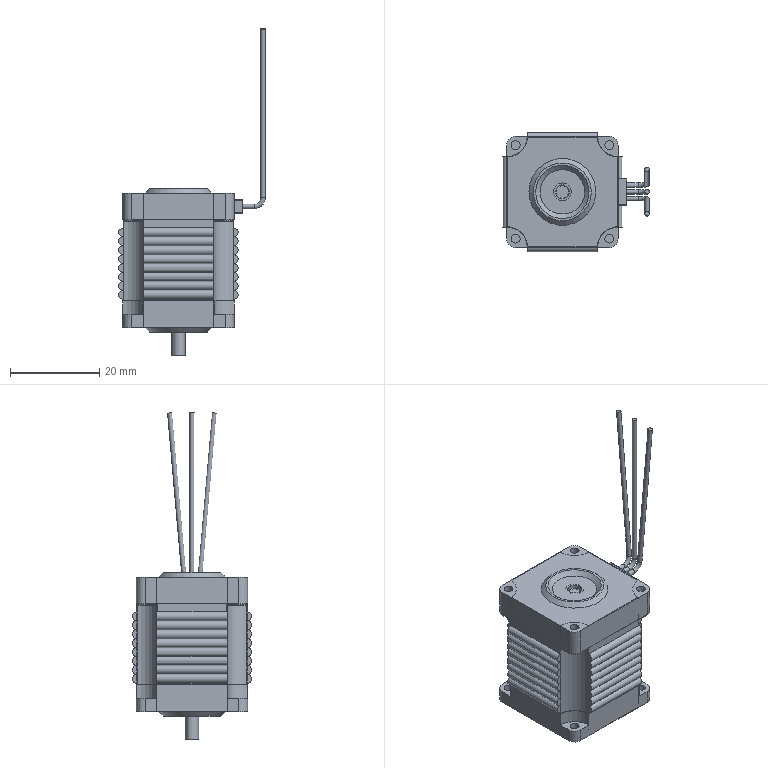Assembly | NX | mm | 8 component files | 8 solids | 300 faces | box 32.9 x 26.8 x 73.5 mm | volume 2197 mm3 | plane 145 | cylinder 119 | cone 19 | torus 10 | sphere 7 | commonest cylinder face diameters 2 x40 0.2 x23 9.2 x16 4 x13 1 x9 3 x5 9.4 x4 9 x4
Bill of materials:
unnamed part 1 | 1 |  | Flat annular ring with a central circular through-hole and small chamfers on the outer edges of both faces.
unnamed part 2 | 1 |  | Open square tray or cup on a rounded-square base flange. There is a through-hole at each of the four corners, and the walls have concave quarter-round notches at the corners next to the holes. The floor has a recessed circular annular groove and a small raised central boss with a through-hole. The underside has a shallow circular chamfered protrusion.
unnamed part 3 | 1 |  | Rounded-square solid block with a through-hole at each of the four corners. On one face is a raised truncated-cone circular boss with an annular recess and a central hole. A small rectangular protrusion sticks out from one side face; it has a recessed rectangular opening containing three small circular holes.
unnamed part 4 | 1 |  | Plain solid straight cylindrical rod with flat ends. It is long compared to its diameter.
unnamed part 5 | 1 |  | Hollow square tube-like shell, open at both ends. Each corner has a concave scalloped channel running its full height. A set of evenly spaced horizontal rounded ribs or rolls covers the middle band of each face, and thin lobed tabs or flanges stick out at the corners near one end.
unnamed part 6 | 3 |  | Thin solid round wire or rod with one bend of roughly 90 degrees near one end, giving a long straight leg and a short straight leg.
Mates:
1. parallel | Stepper_Front 1 face | Stepper_Mid 1 face
2. distance | Stepper_Front 1 face | Stepper_Mid 1 face
3. fix | Stepper_Front 1 component
4. touch align | Stepper_Front 1 face | Stepper_Washer 1 face
5. distance | Stepper_Front 1 face | Stepper_Washer 1 face
6. parallel | Stepper_Back 1 face | Stepper_Front 1 face
7. touch align | Stepper_Mid 1 face | Stepper_Back 1 face
8. touch align | Stepper_Back 1 face | Stepper_Shaft 1 face
9. distance | Stepper_Back 1 face | Stepper_Shaft 1 face
10. distance | Stepper_Mid 1 face | Stepper_Front 1 face
11. concentric | Stepper_Wire 3 edge | Stepper_Back 1 edge
12. touch align | Stepper_Back 1 face | Stepper_Wire 2 face
13. concentric | Stepper_Wire 2 edge | Stepper_Back 1 edge
14. distance | Stepper_Back 1 face | Stepper_Mid 1 face
15. touch align | Stepper_Wire 1 face | Stepper_Back 1 face
16. concentric | Stepper_Wire 1 edge | Stepper_Back 1 edge
17. distance | Stepper_Front 1 face | Stepper_Mid 1 face
18. touch align | Stepper_Back 1 face | Stepper_Mid 1 face